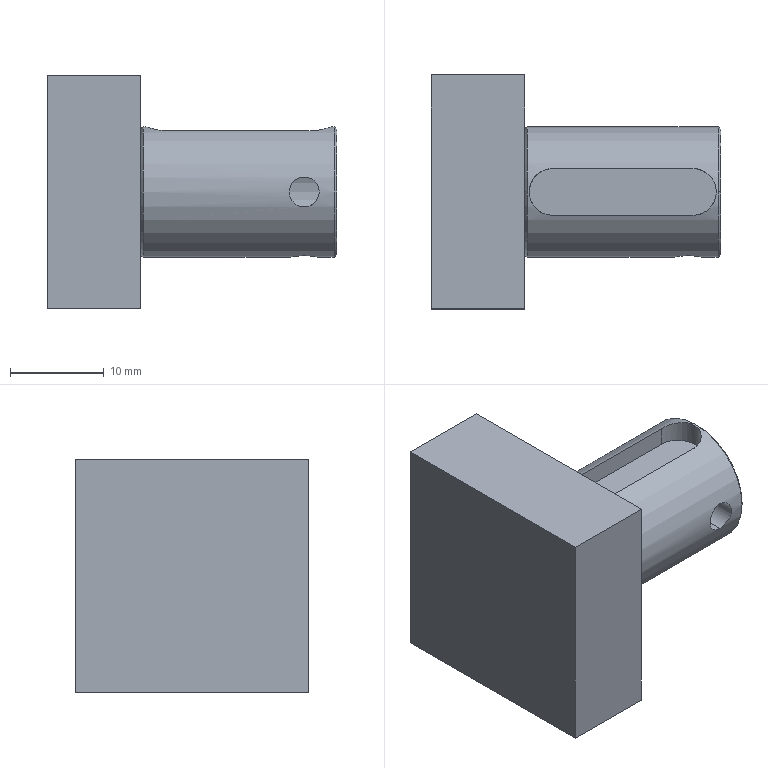CAM job | Mastercam | mm | 9 operations | part box 31 x 25 x 25
1. Facing | 20 - 63 平铣刀
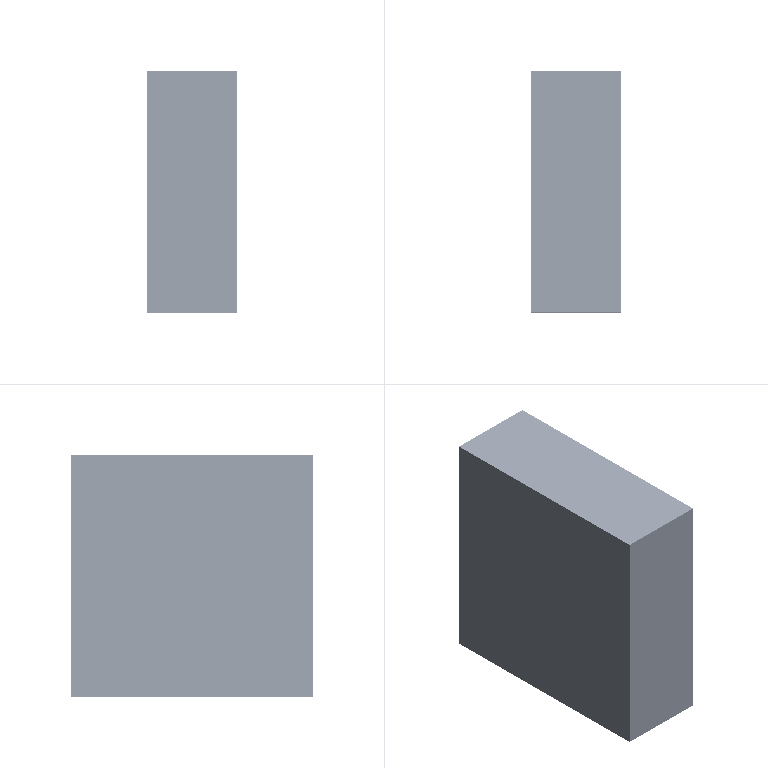2. 3D High Speed (Dynamic OptiRough) | 8 - 8 平铣刀
3. Contour (Remachining) | 2 - 2 平铣刀
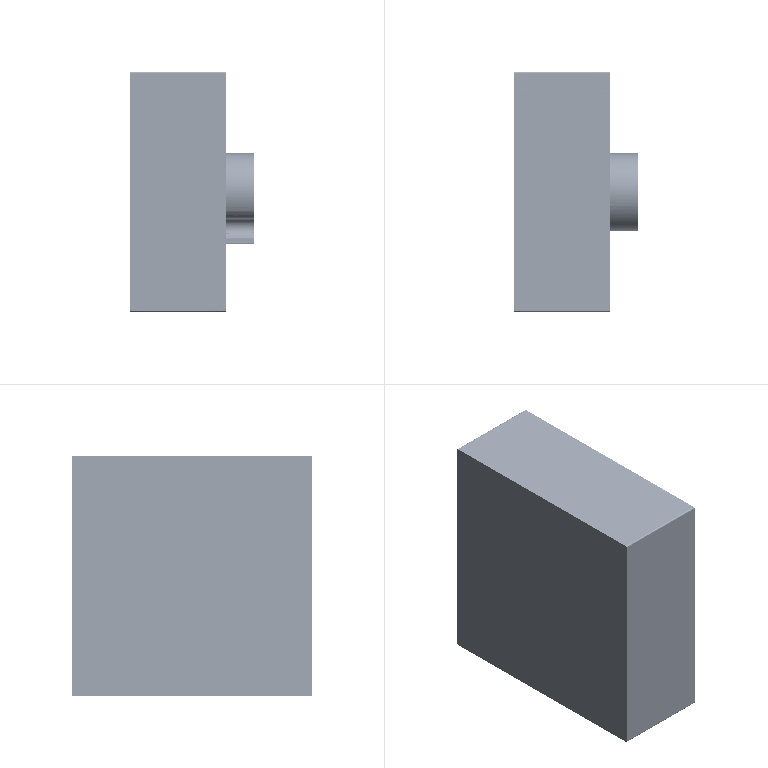4. Contour (Ramp) | 1 - 1 平铣刀
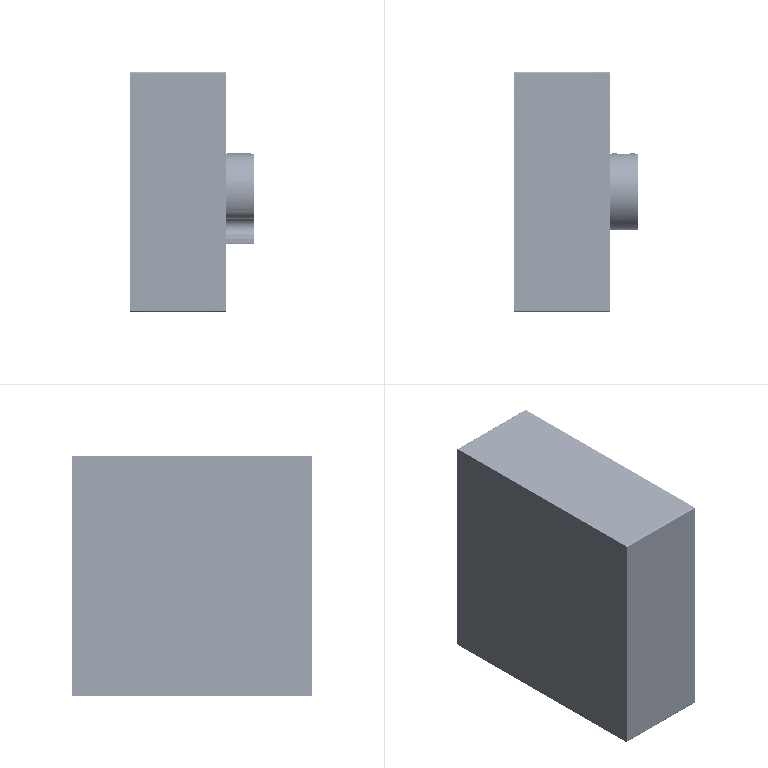5. 2D High Speed (2D Area Mill) | 2 - 2 平铣刀
6. Contour (2D) | 8 - 8 平铣刀
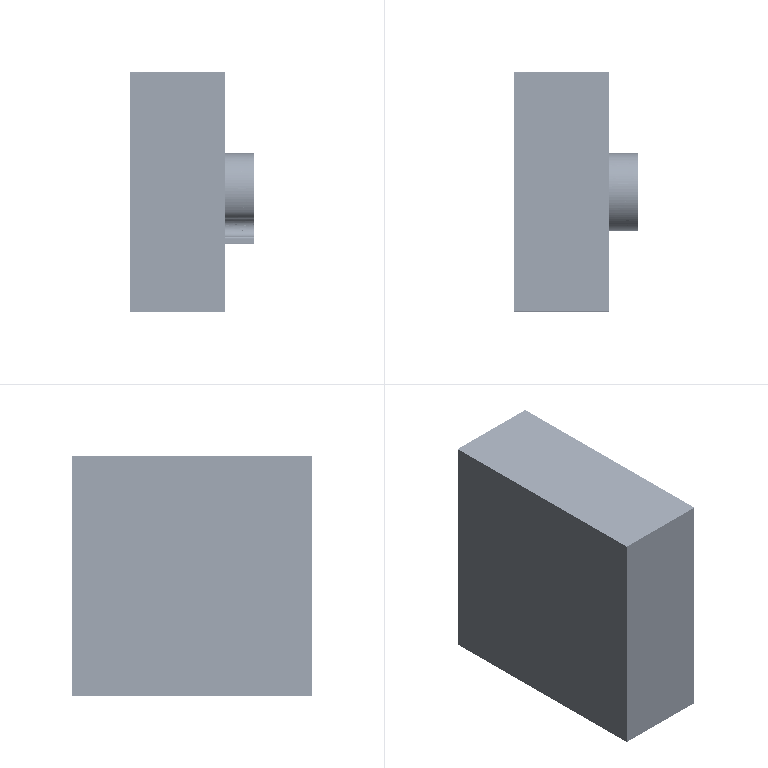7. Contour (2D chamfer) | 7 - 4 倒角刀
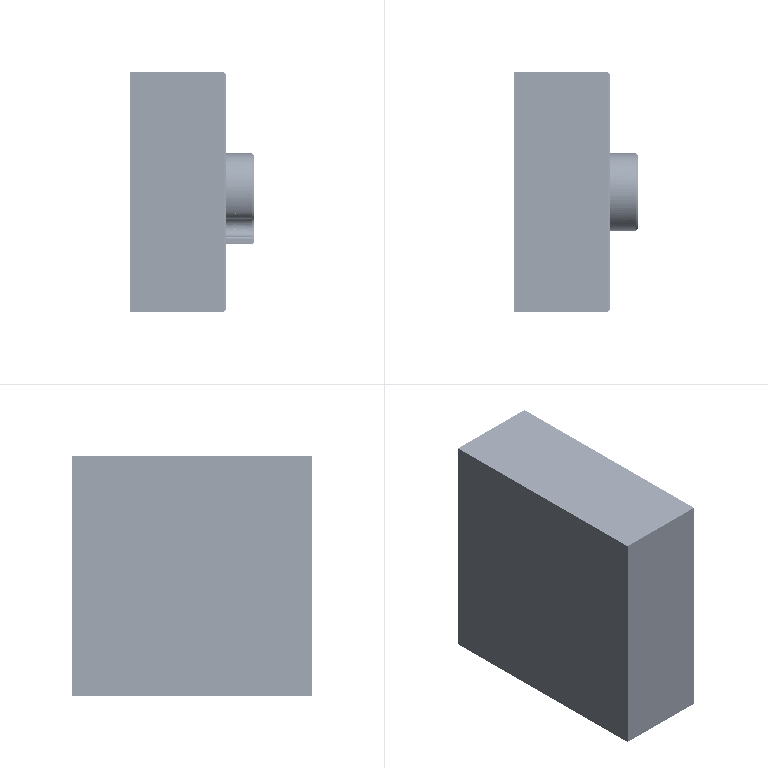8. Contour (Ramp) | 3 - 3 平铣刀
9. Drill/Counterbore | 7 - 4 倒角刀